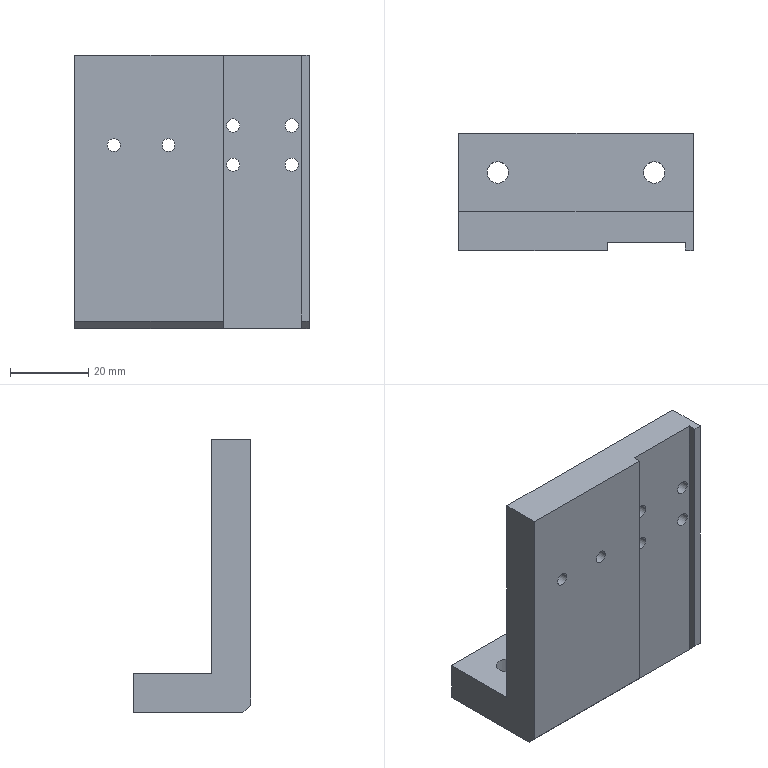Component | SolidWorks | P-SLJ-004-3_P-SLJ-004-001-1 | 1 solid | 42 faces | box 60 x 30 x 70 mm | volume 49922 mm3 | cylinder 24 | plane 18 | commonest cylinder face diameters 6 x8 3.4 x8 3.3 x4 5.5 x4 | material A3
build123d program:
from build123d import *

# Parameters (mm, degrees)
EXTRUDE1_DEPTH                                       = 30
M5_CLEARANCE_HOLE1_D                                 = 5.5
SKETCH4_W                                            = 20
SKETCH4_H                                            = 2
EXTRUDE2_DEPTH                                       = 82.854
CBORE_FOR_M3_HEXAGON_SOCKET_HEAD_CAP_SCR_D           = 3.4
CBORE_FOR_M3_HEXAGON_SOCKET_HEAD_CAP_SCR_CBORE_D     = 6
CBORE_FOR_M3_HEXAGON_SOCKET_HEAD_CAP_SCR_CBORE_DEPTH = 3.4
M4_TAPPED_HOLE2_D                                    = 3.3
CHAMFER1_SIZE                                        = 2


with BuildPart() as part:
    # Sketch1 → Extrude1 (new, symmetric)
    with BuildSketch(Plane.XY):
        Polygon((0, 0), (70, 0), (70, 10), (10, 10), (10, 30), (0, 30), align=None)
    extrude(amount=EXTRUDE1_DEPTH, both=True)

    # M5 Clearance Hole1 (through all)
    with Locations(Plane(origin=(10, 0, 0), x_dir=(0, 0, -1), z_dir=(1, 0, 0))):
        with Locations((-20, 20), (20, 20)):
            Hole(M5_CLEARANCE_HOLE1_D / 2)

    # Sketch4 → Extrude2 (cut, through all)
    with BuildSketch(Plane(origin=(70, 0, 0), x_dir=(0, 0, -1), z_dir=(1, 0, 0))):
        with Locations((18, 1)):
            Rectangle(SKETCH4_W, SKETCH4_H)
    extrude(amount=-EXTRUDE2_DEPTH, mode=Mode.SUBTRACT)

    # CBORE for M3 Hexagon socket head cap scr (through all)
    with Locations(Plane(origin=(0, 10, 0), x_dir=(1, 0, 0), z_dir=(0, 1, 0))):
        with Locations((42, 25.5), (52, 25.5), (52, 10.5), (42, 10.5)):
            CounterBoreHole(CBORE_FOR_M3_HEXAGON_SOCKET_HEAD_CAP_SCR_D / 2, CBORE_FOR_M3_HEXAGON_SOCKET_HEAD_CAP_SCR_CBORE_D / 2, CBORE_FOR_M3_HEXAGON_SOCKET_HEAD_CAP_SCR_CBORE_DEPTH)

    # M4 Tapped Hole2 (through all)
    with Locations(Plane(origin=(0, 10, 0), x_dir=(1, 0, 0), z_dir=(0, 1, 0))):
        with Locations((47, -6), (47, -20)):
            Hole(M4_TAPPED_HOLE2_D / 2)

    # Chamfer1
    chamfer1_edges = [part.edges().sort_by_distance(p)[0] for p in [
        (0, 0, -29),
        (0, 0, 11),
    ]]
    chamfer(chamfer1_edges, length=CHAMFER1_SIZE)


solid = part.part

# Placed as in the assembly
solid = solid.moved(Location((-219.5, -33, 1235.634), (0, -90, 0)))